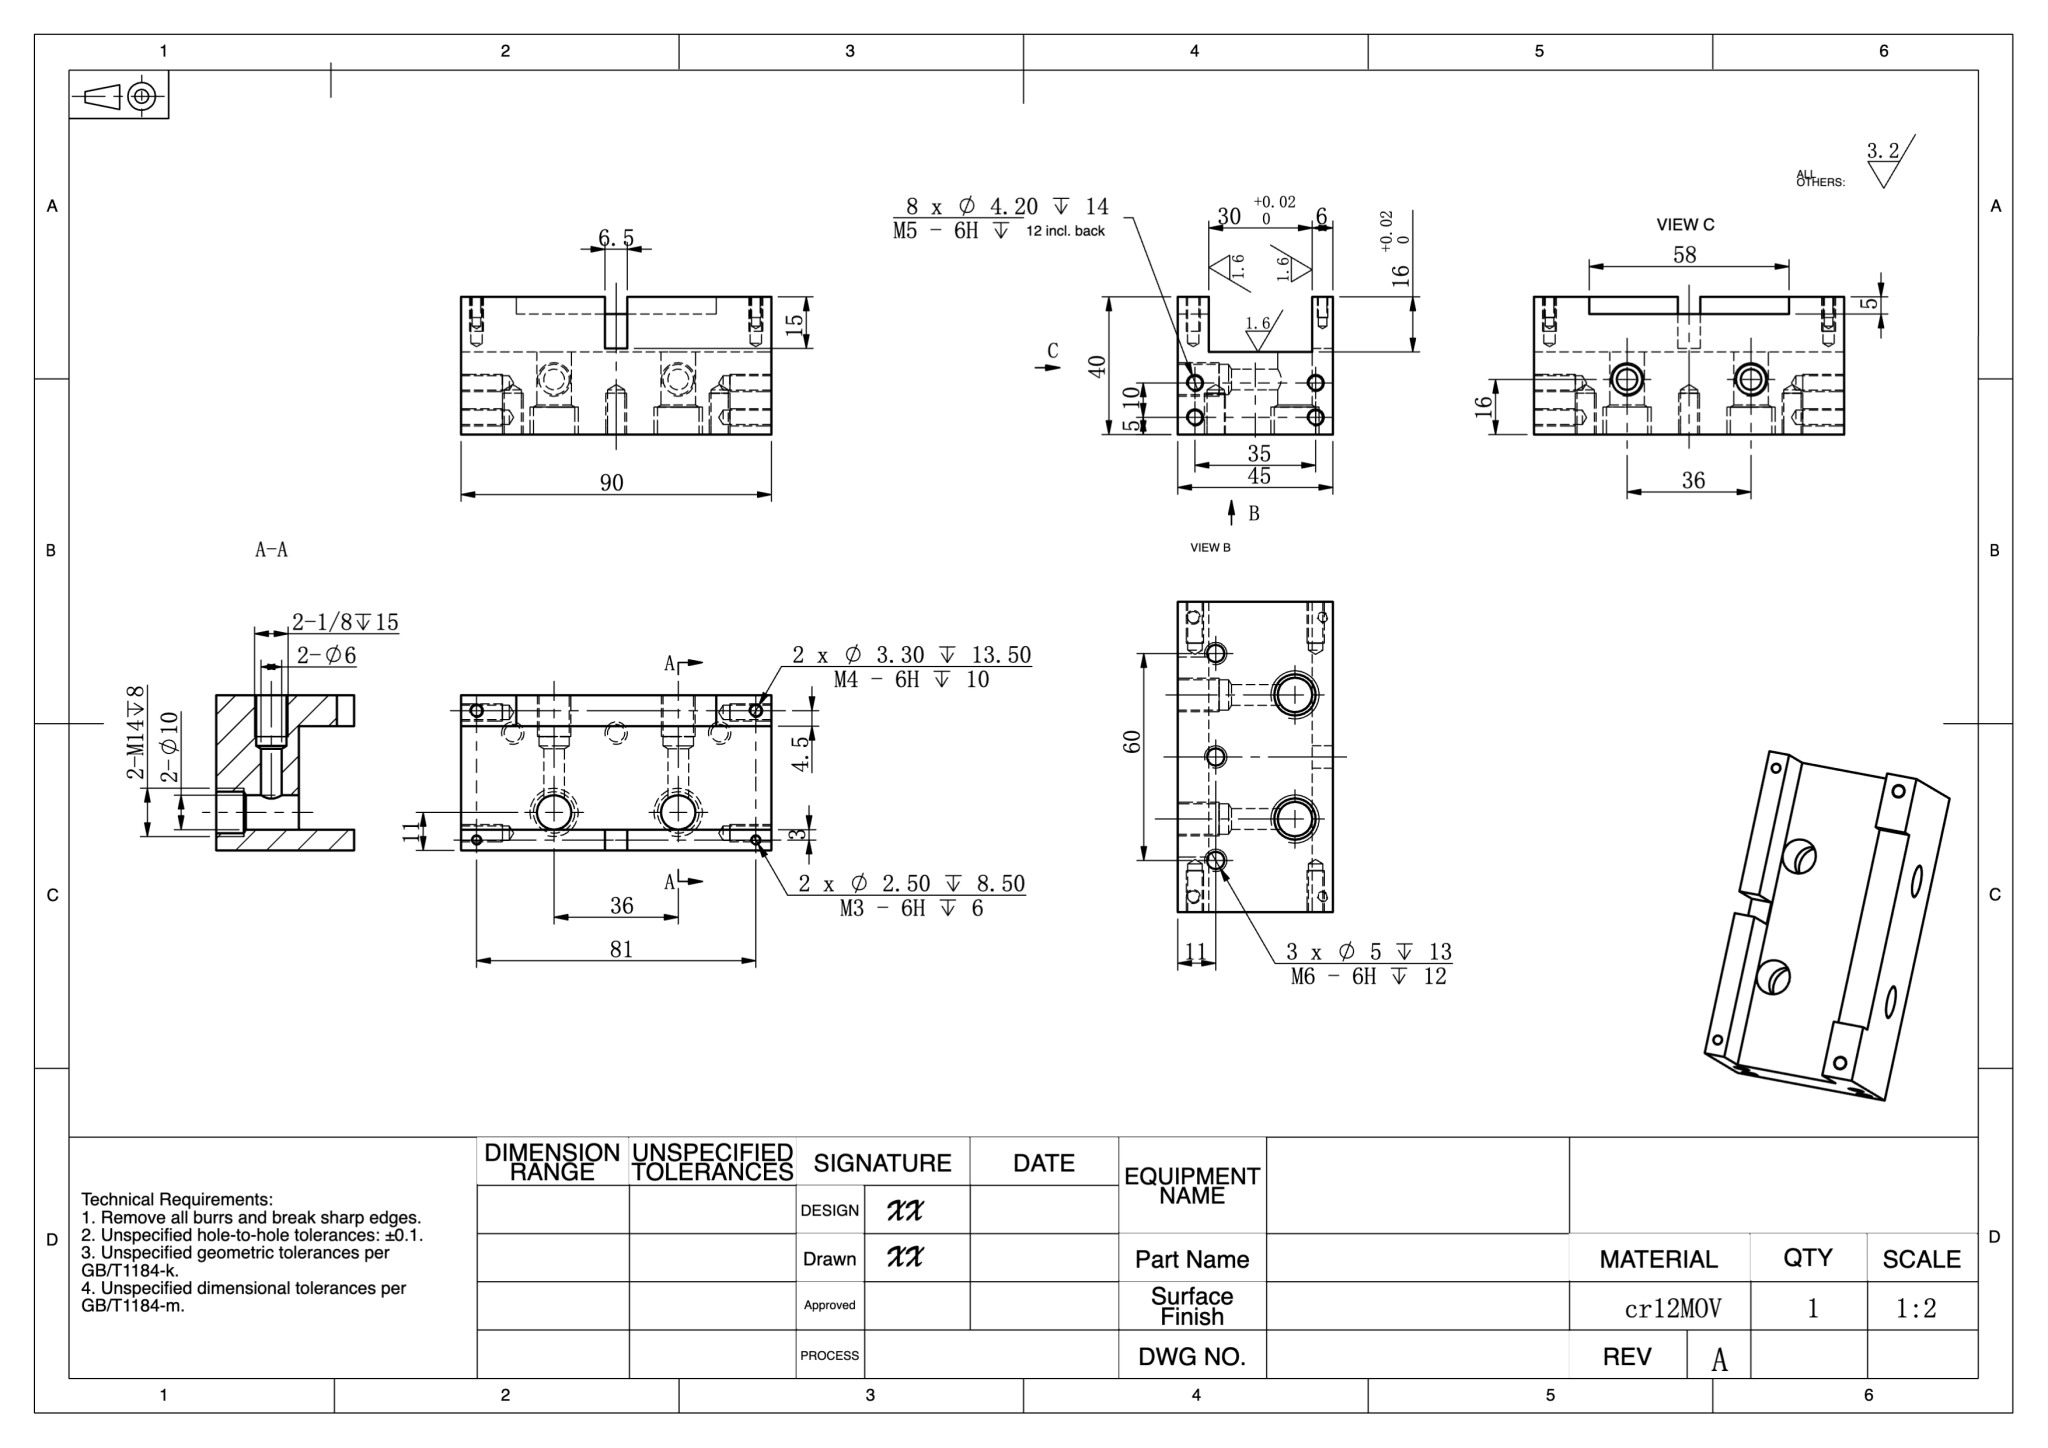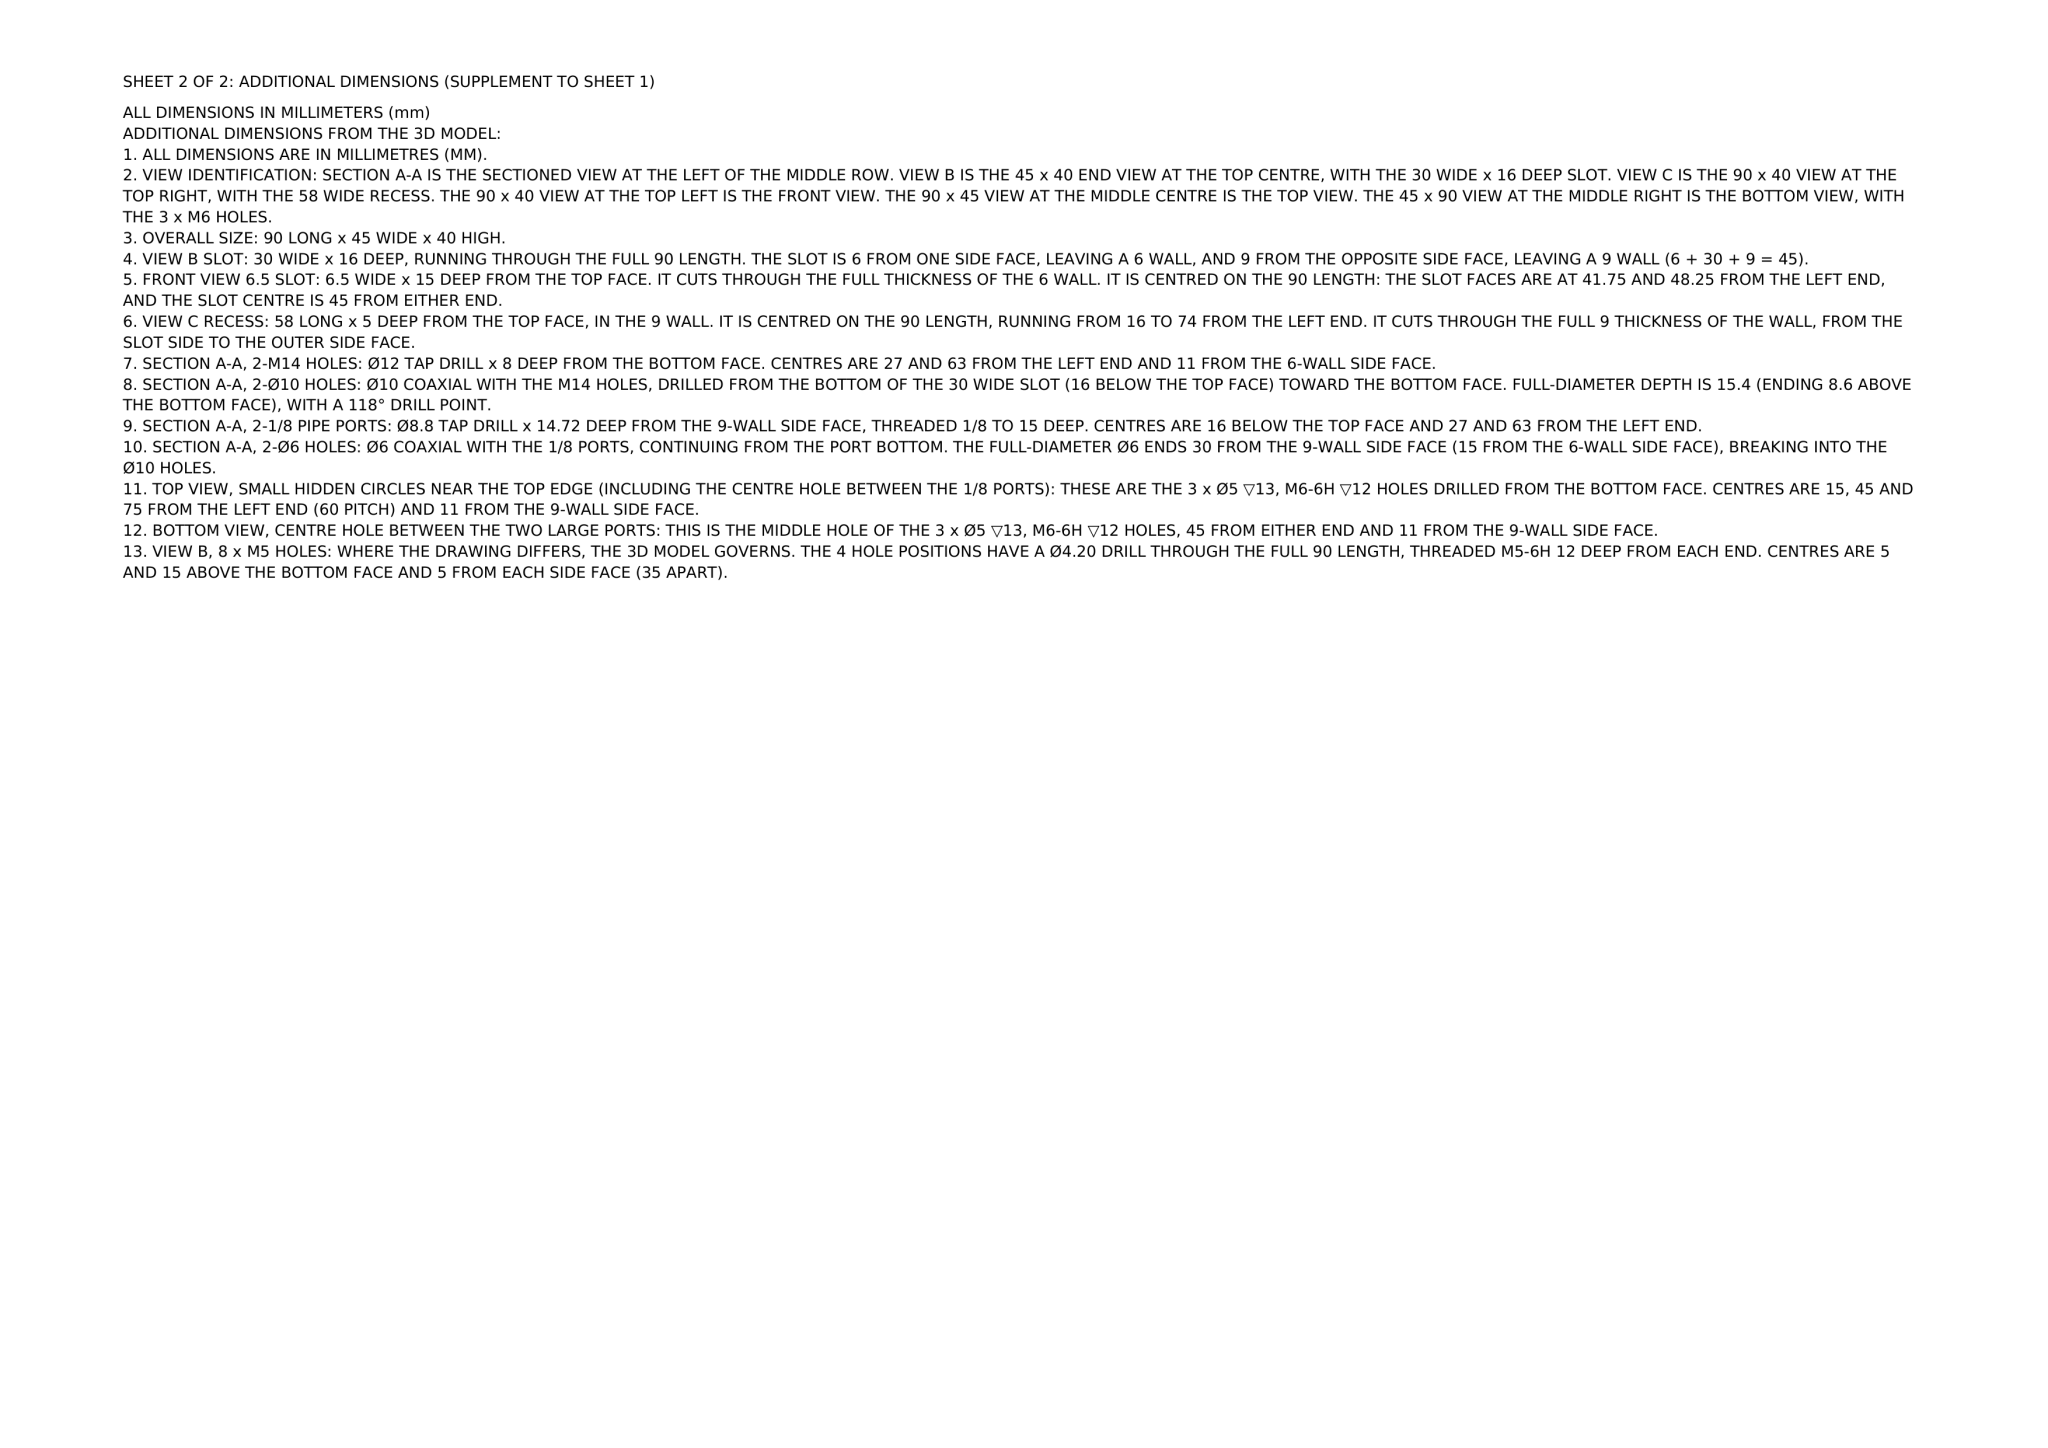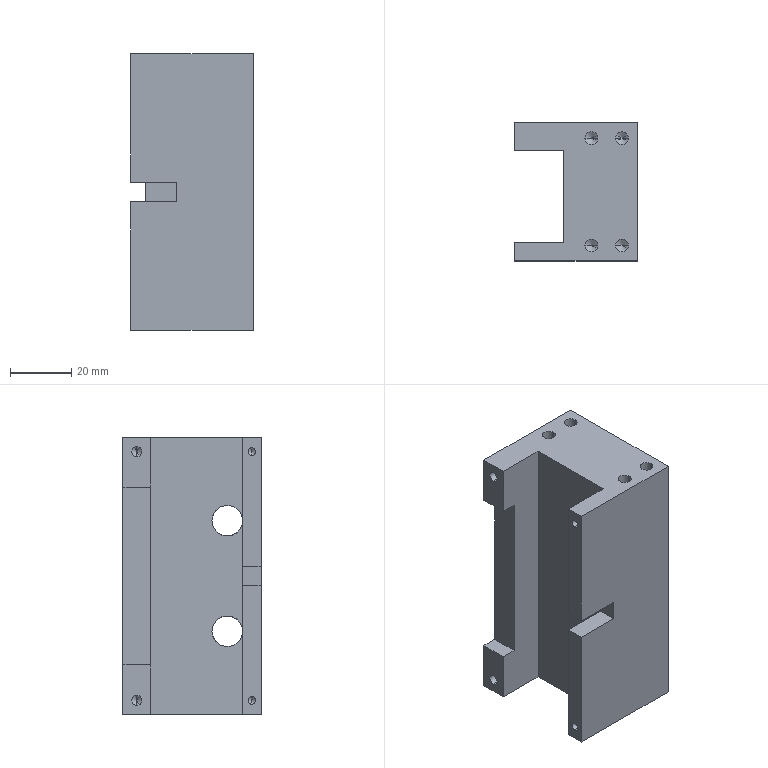Part | NX | mm | C-Channel Mounting Block | 1 solid | 102 faces | box 40 x 45 x 90 mm | volume 105909 mm3 | cylinder 46 | cone 38 | plane 18 | commonest cylinder face diameters 4.2 x16 5 x6 2.5 x4 3.3 x4 8.8 x4 6 x4 12 x4 10 x4